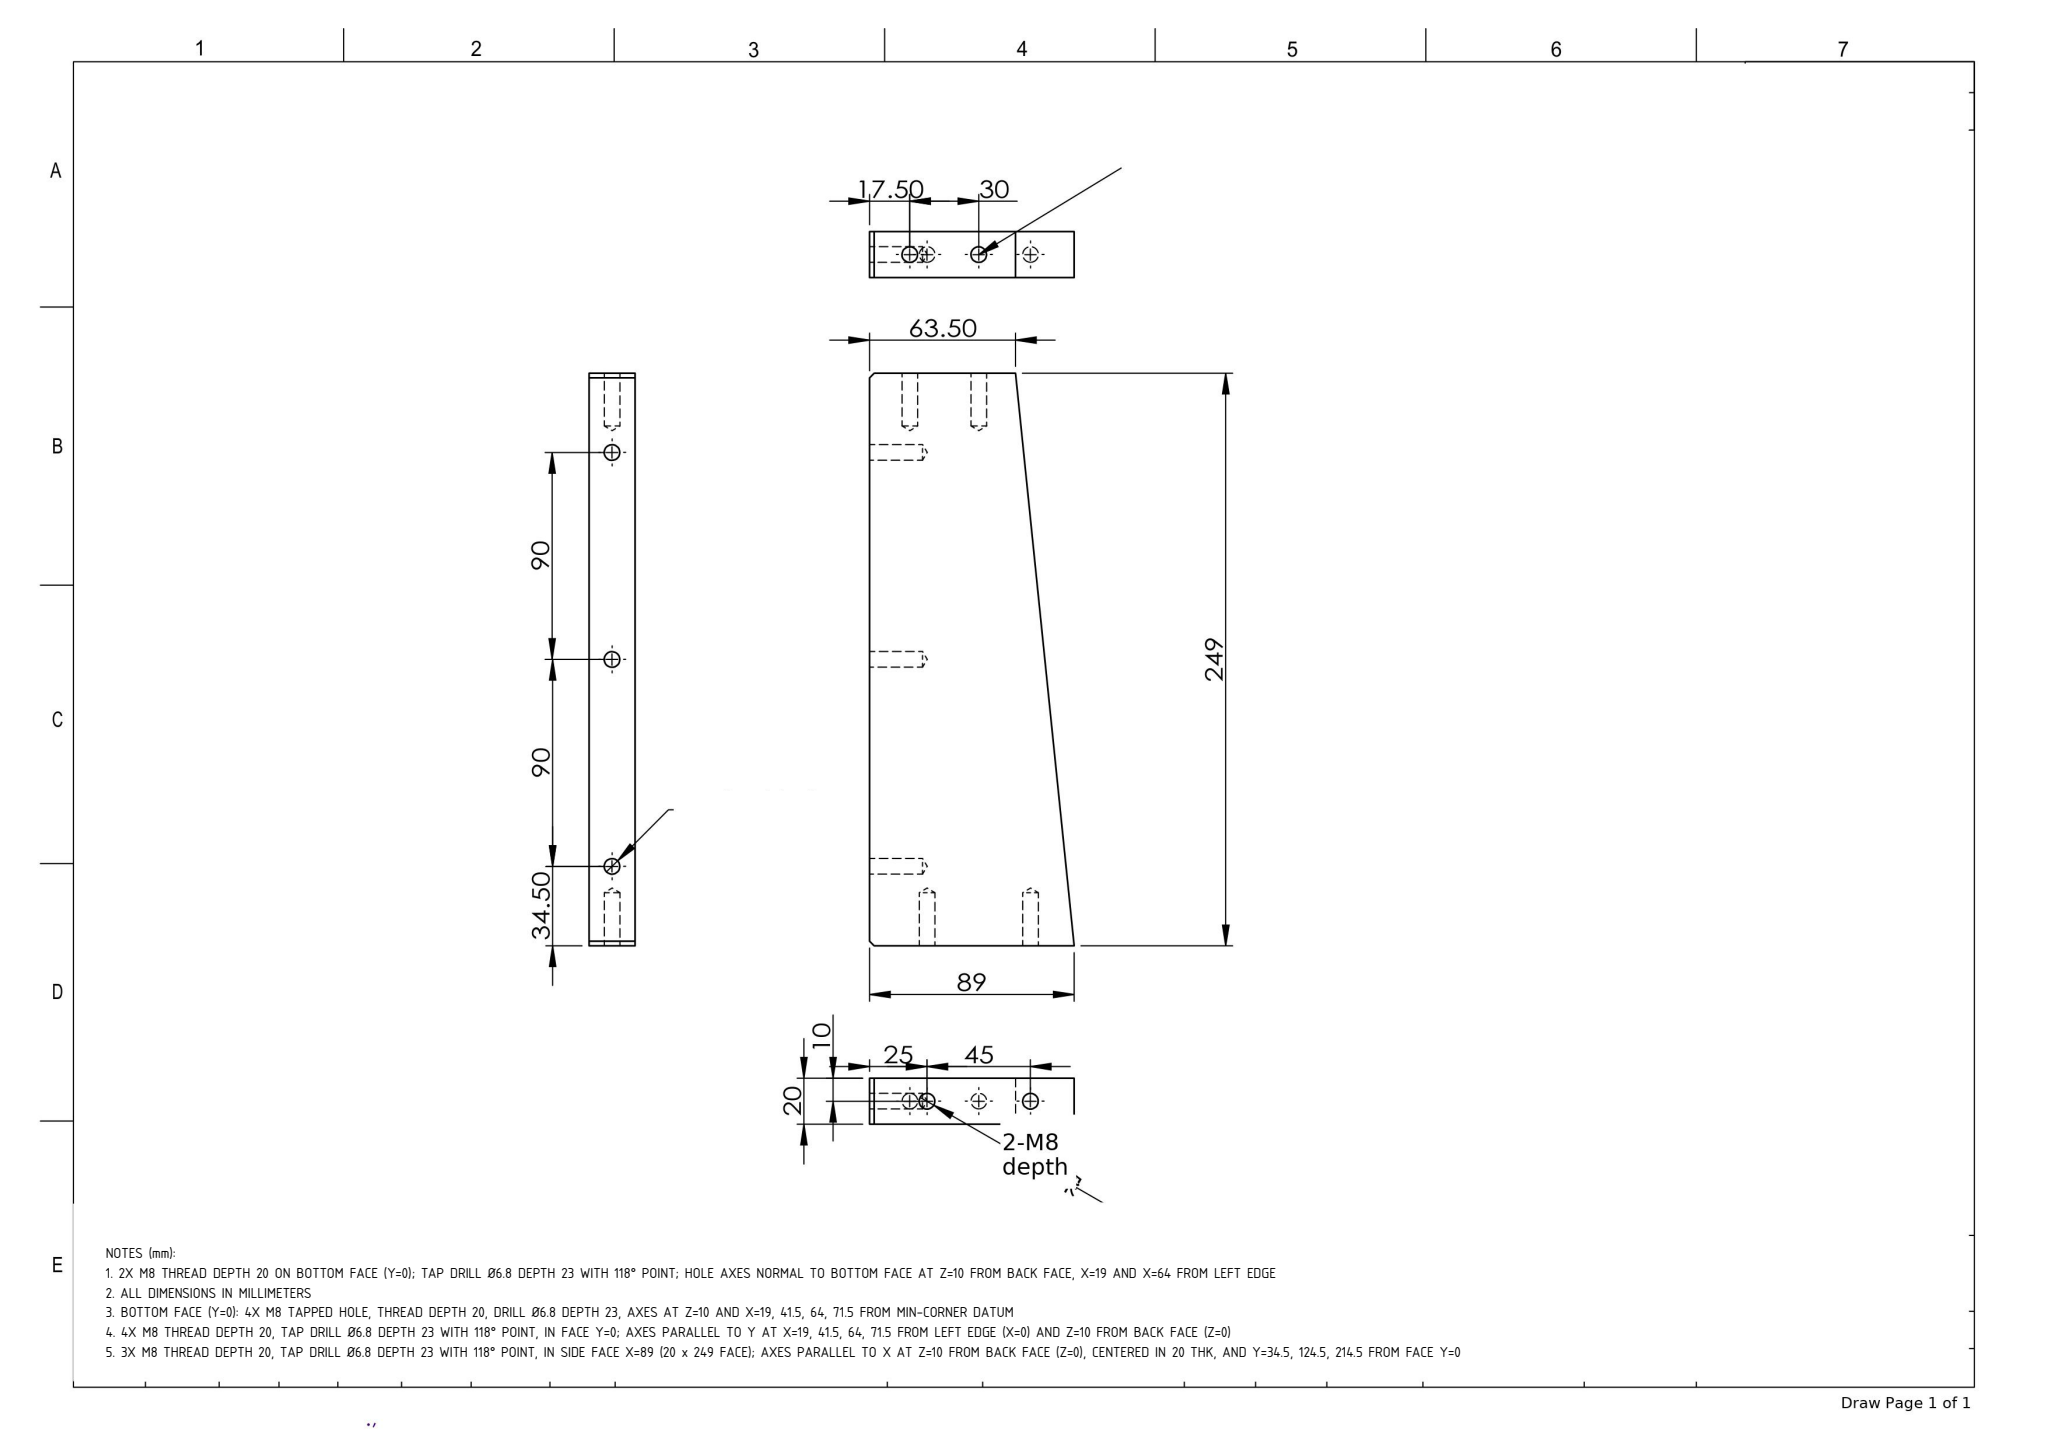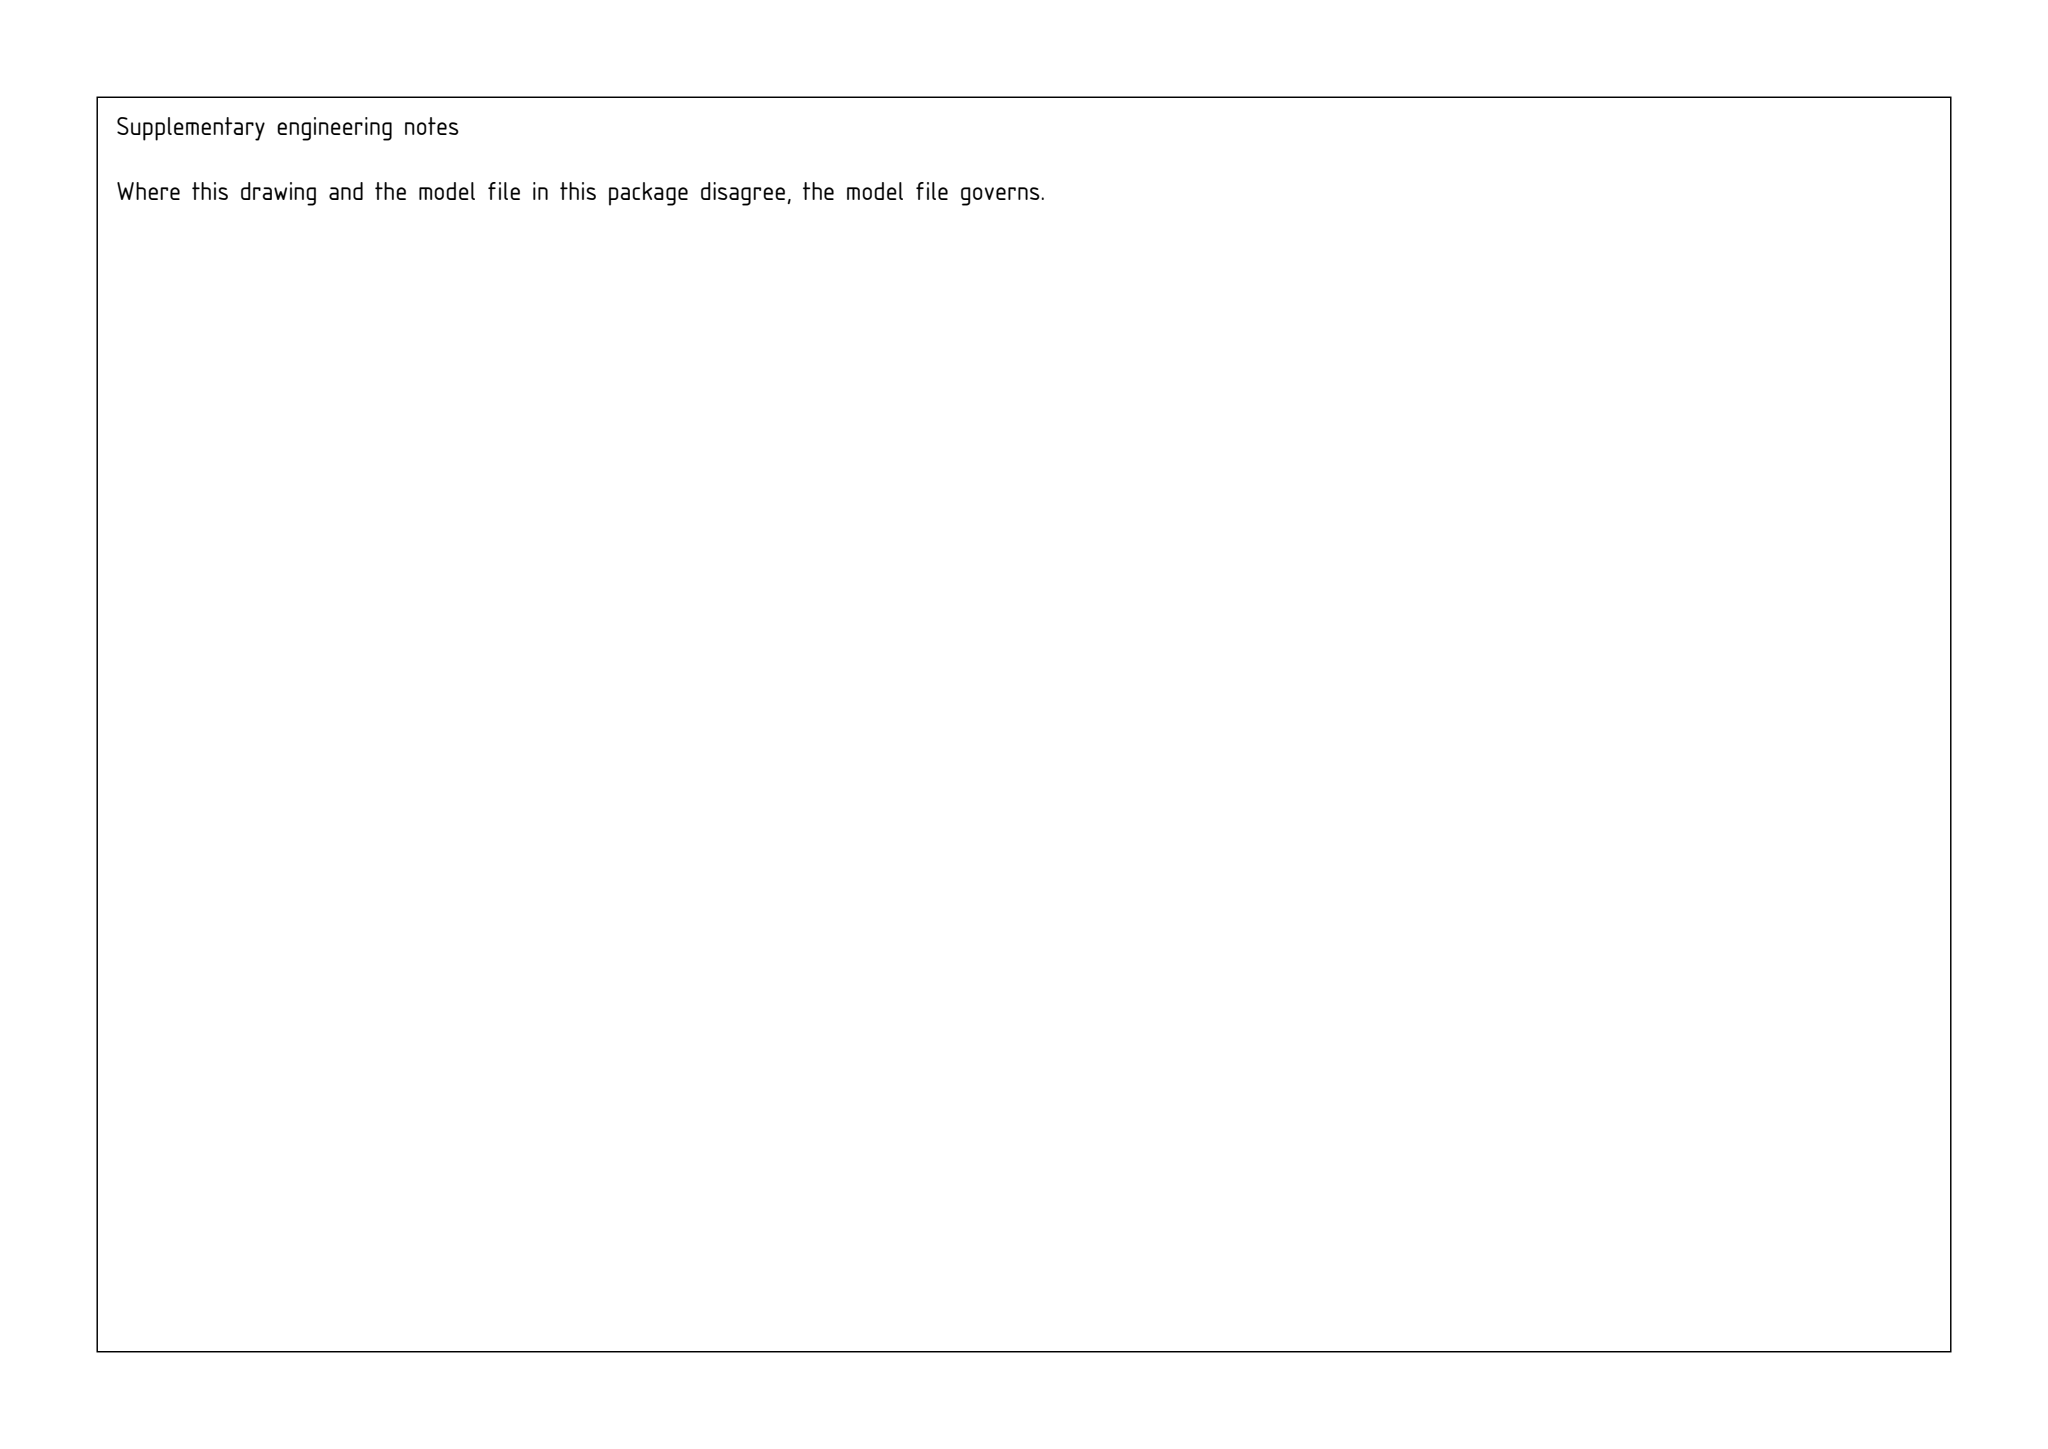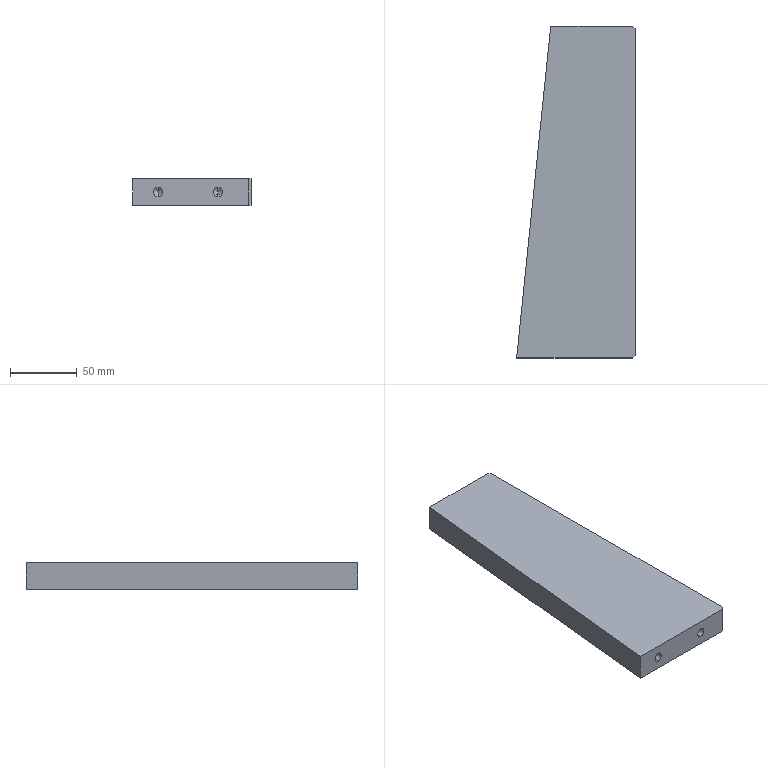Part | SolidWorks | mm | 1 solid | 36 faces | box 89 x 249 x 20 mm | volume 373625 mm3 | cylinder 14 | cone 14 | plane 8 | commonest cylinder face diameters 6.8 x14
Drawing notes:
2X M8 THREAD DEPTH 20 ON BOTTOM FACE (Y=0); TAP DRILL Ø6.8 DEPTH 23 WITH 118° POINT; HOLE AXES NORMAL TO BOTTOM FACE AT Z=10 FROM BACK FACE, X=19 AND X=64 FROM LEFT EDGE | from the solid: cylinders [6.8,'y',[19.0,null,10.0],23.0] and [6.8,'y',[64.0,null,10.0],23.0]; cones [118.0, ref_dia 6.8]
ALL DIMENSIONS IN MILLIMETERS | from the solid: STEP model facts units (mm), bbox_xyz 89.0 x 249.0 x 20.0
BOTTOM FACE (Y=0): 4X M8 TAPPED HOLE, THREAD DEPTH 20, DRILL Ø6.8 DEPTH 23, AXES AT Z=10 AND X=19, 41.5, 64, 71.5 FROM MIN-CORNER DATUM | from the solid: cylinders dia 6.8 axis y at [19,null,10], [41.5,null,10], [64,null,10], [71.5,null,10], length 23; cones 118° ref dia 6.8
4X M8 THREAD DEPTH 20, TAP DRILL Ø6.8 DEPTH 23 WITH 118° POINT, IN FACE Y=0; AXES PARALLEL TO Y AT X=19, 41.5, 64, 71.5 FROM LEFT EDGE (X=0) AND Z=10 FROM BACK FACE (Z=0) | from the solid: cylinders dia 6.8 axis y at pos (19,null,10),(41.5,null,10),(64,null,10),(71.5,null,10) length 23; cones 118° ref dia 6.8; axis_planes y=0, z=0
3X M8 THREAD DEPTH 20, TAP DRILL Ø6.8 DEPTH 23 WITH 118° POINT, IN SIDE FACE X=89 (20 x 249 FACE); AXES PARALLEL TO X AT Z=10 FROM BACK FACE (Z=0), CENTERED IN 20 THK, AND Y=34.5, 124.5, 214.5 FROM FACE Y=0 | from the solid: cylinders dia 6.8 axis x at pos (null,34.5,10),(null,124.5,10),(null,214.5,10) length 23; axis_planes x=89, z=0 and z=20